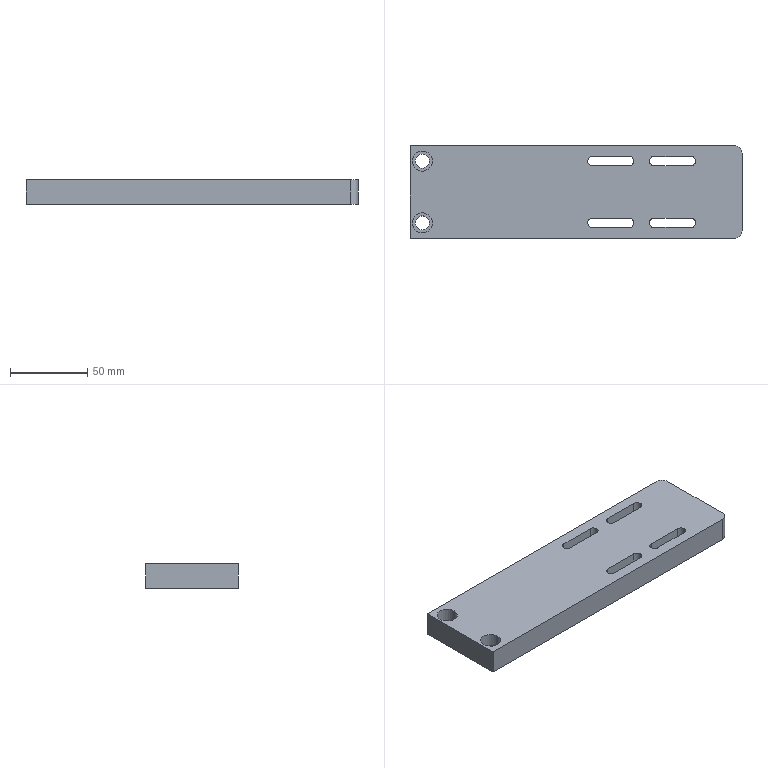CAM job | Mastercam | mm | 2 operations | part box 215 x 60 x 16
1. Facing | 24 - 100 平铣刀
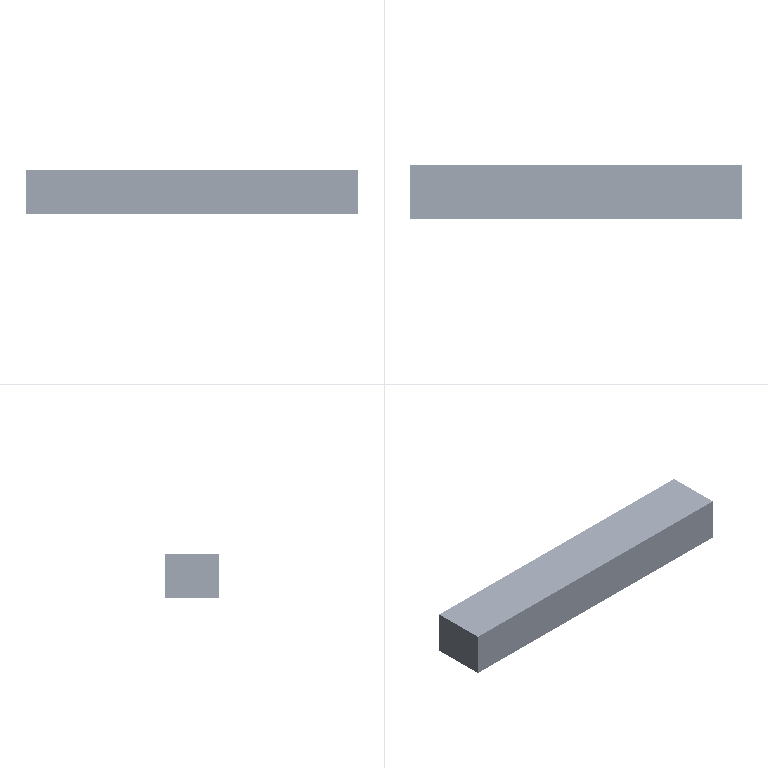2. Contour (2D chamfer) | 7 - 4 倒角刀